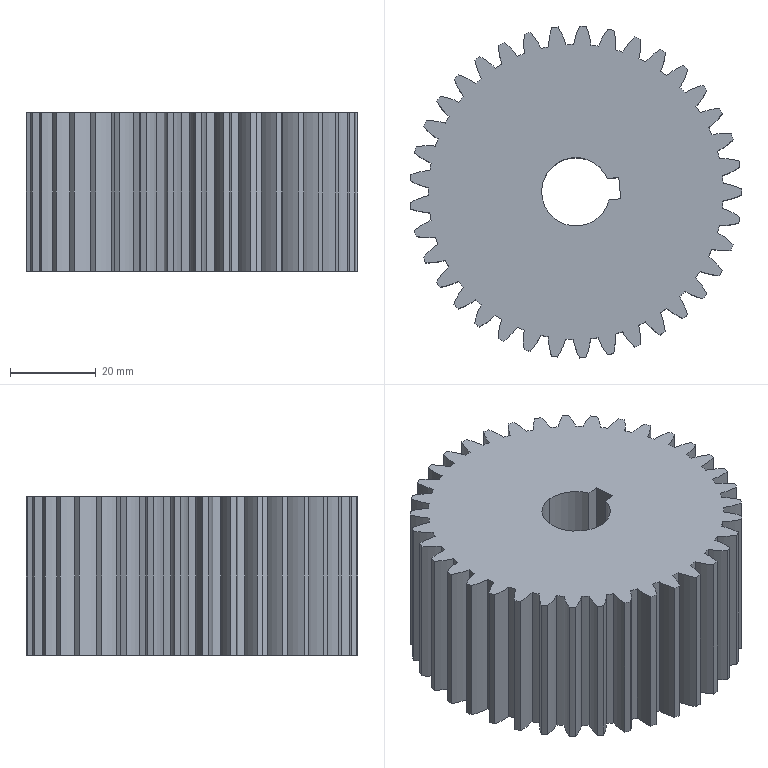Component | SolidWorks | spur gear_gb-1 | 1 solid | 160 faces | box 77.52 x 77.58 x 37 mm | volume 148158 mm3 | cylinder 155 | plane 5 | commonest cylinder face diameters 29.6 x78 77.6 x37 68.998 x37 16 x3
build123d program:
from build123d import *

# Parameters (mm, degrees)
BASPROSKE_W     = 37
BASPROSKE_H     = 38.8
TOOTHCUT_DEPTH  = 67.181
TEETHCUTS_COUNT = 37
TEETHCUTS_ANGLE = 350.27
BORSKE_R        = 8
BORE_DEPTH      = 50
KEYSKE_W        = 5
KEYSKE_H        = 10.3
KEYWAY_DEPTH    = 50


with BuildPart() as part:
    # BasProSke → Base-Revolve (revolve)
    with BuildSketch(Plane(origin=(0, 0, 0), x_dir=(1, 0, 0), z_dir=(0, 1, 0)), mode=Mode.PRIVATE) as base_revolve_sk:
        with Locations((18.5, 19.4)):
            Rectangle(BASPROSKE_W, BASPROSKE_H)
    revolve(base_revolve_sk.sketch.rotate(Axis((-10, 0, 0), (1, 0, 0)), 180), axis=Axis((-10, 0, 0), (1, 0, 0)))

    # TooCutSke → ToothCut (cut, through all)
    with BuildSketch(Plane(origin=(0, 0, 0), x_dir=(0, 0, -1), z_dir=(1, 0, 0))):
        with BuildLine():
            ThreePointArc((0.8916, 34.487), (0, 34.499), (-0.8916, 34.487))
            ThreePointArc((-0.8916, 34.487), (-1.572, 36.679), (-2.583, 38.739))
            ThreePointArc((-2.583, 38.739), (0, 38.825), (2.583, 38.739))
            ThreePointArc((2.583, 38.739), (1.572, 36.679), (0.8916, 34.487))
        make_face()
    toothcut = extrude(amount=TOOTHCUT_DEPTH, mode=Mode.SUBTRACT)

    # TeethCuts: ToothCut ×37 about axis
    teethcuts_axis = Axis((-10, 0, 0), (1, 0, 0))
    for i in range(1, TEETHCUTS_COUNT):
        add(toothcut.rotate(teethcuts_axis, i * TEETHCUTS_ANGLE / (TEETHCUTS_COUNT - 1)), mode=Mode.SUBTRACT)

    # BorSke → Bore (cut, symmetric)
    with BuildSketch(Plane(origin=(0, 0, 0), x_dir=(0, 0, -1), z_dir=(1, 0, 0))):
        with Locations(Location((0, 0, 0), (0, 0, 180))):
            Circle(BORSKE_R)
    extrude(amount=BORE_DEPTH, both=True, mode=Mode.SUBTRACT)

    # KeySke → Keyway (cut, symmetric)
    with BuildSketch(Plane(origin=(0, 0, 0), x_dir=(0, 0, -1), z_dir=(1, 0, 0))):
        with Locations((0, 5.15)):
            Rectangle(KEYSKE_W, KEYSKE_H)
    extrude(amount=KEYWAY_DEPTH, both=True, mode=Mode.SUBTRACT)


solid = part.part

# Placed as in the assembly
solid = solid.moved(Location((174.299, -234.1, 81.963), (90, 4.802, -90)))